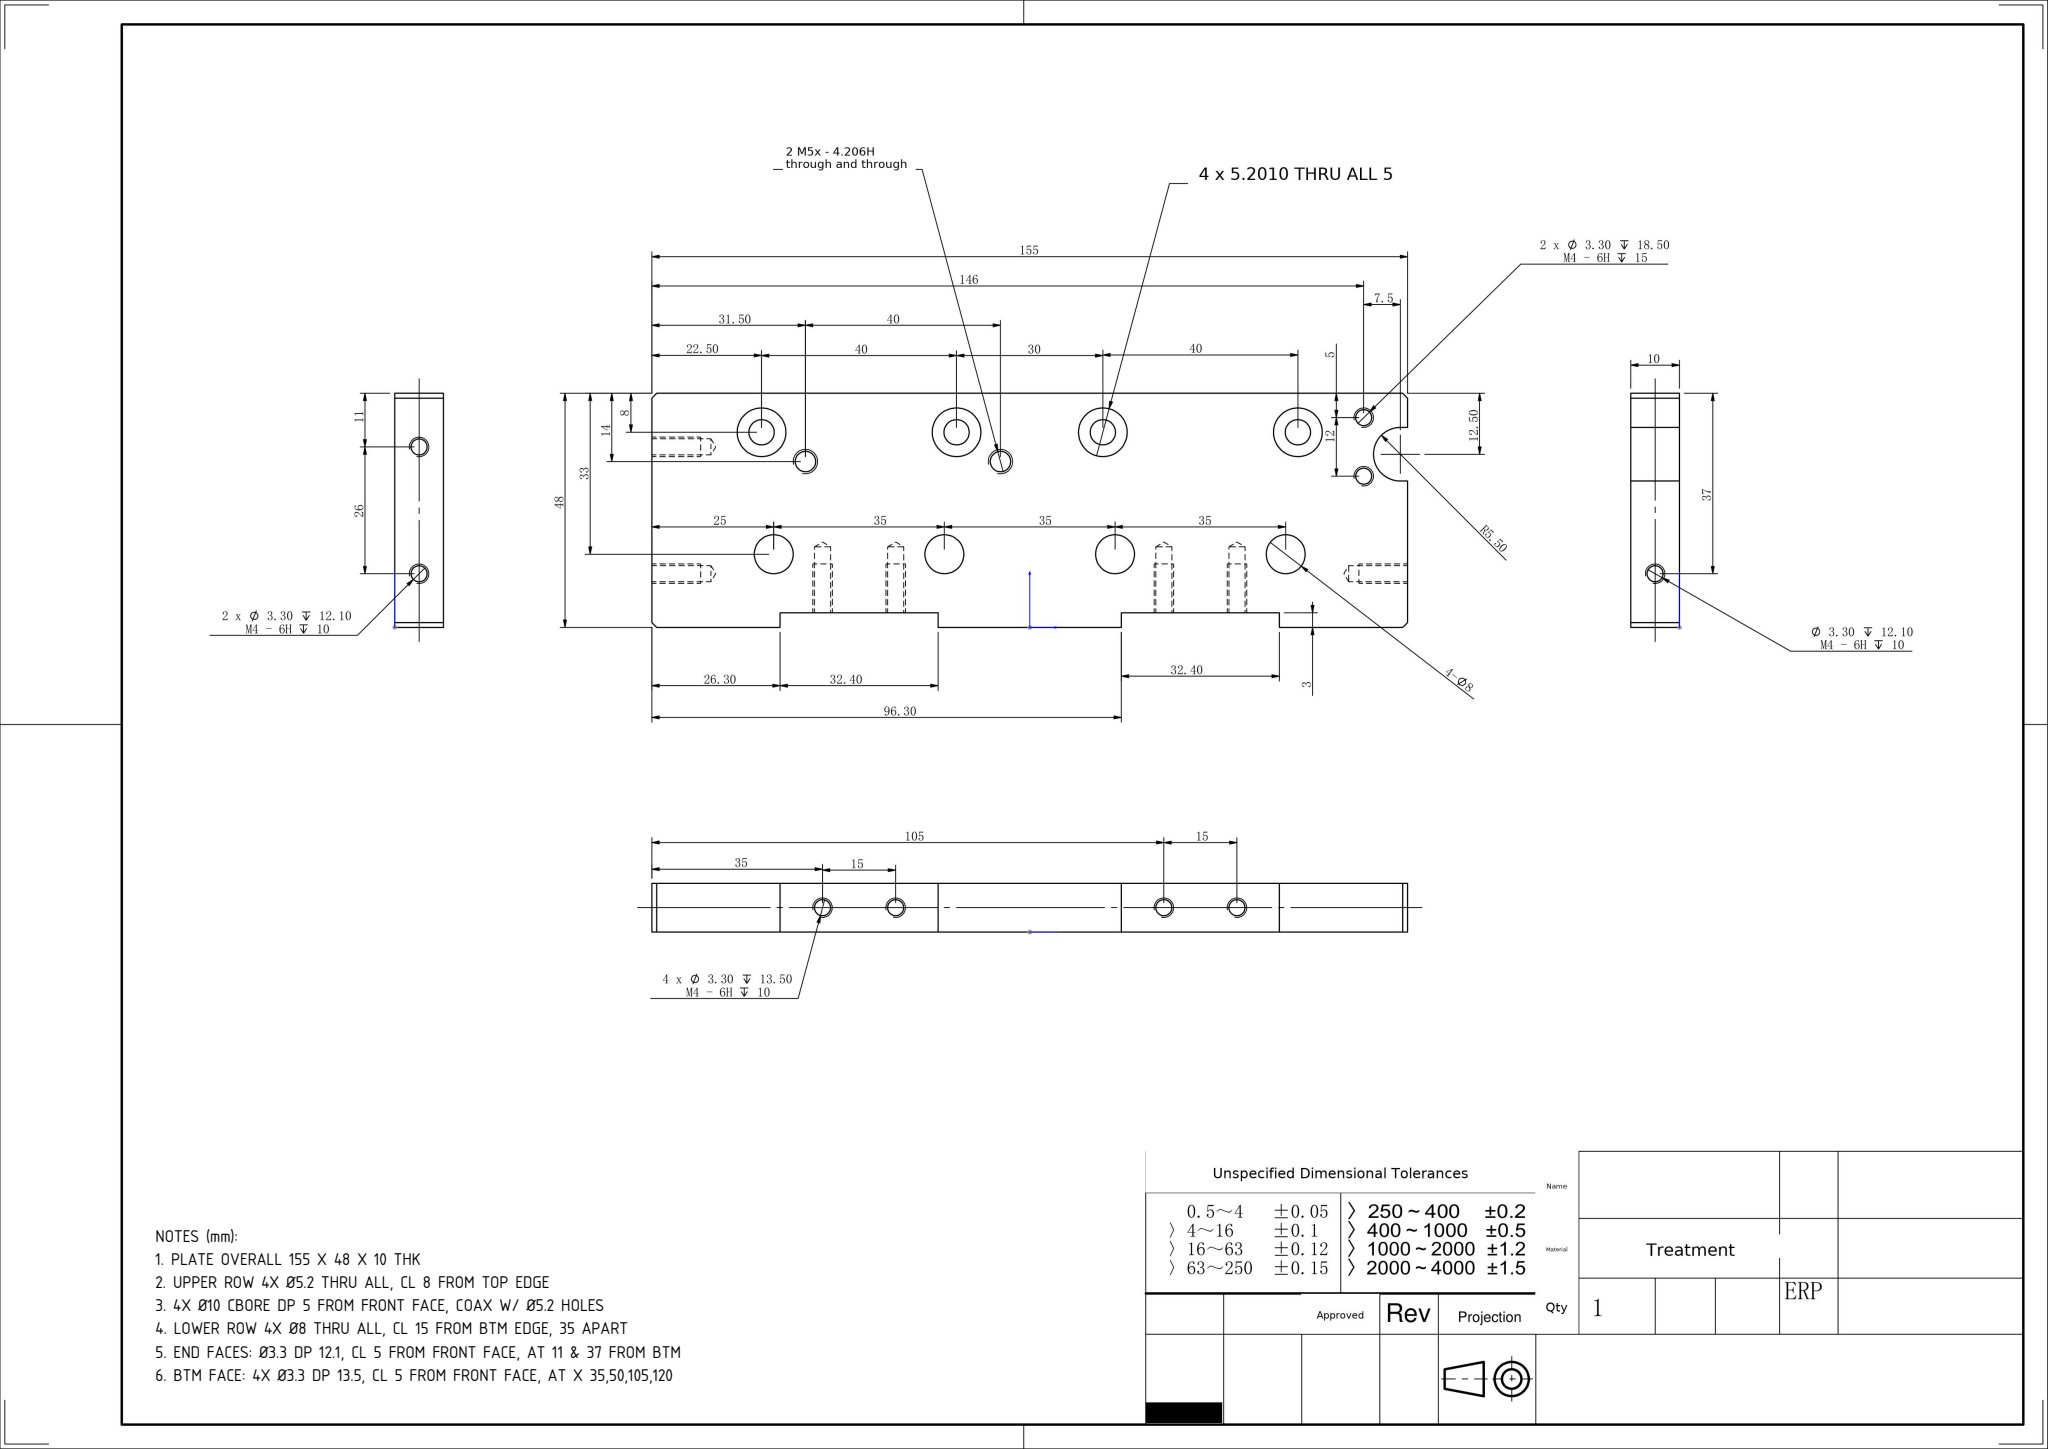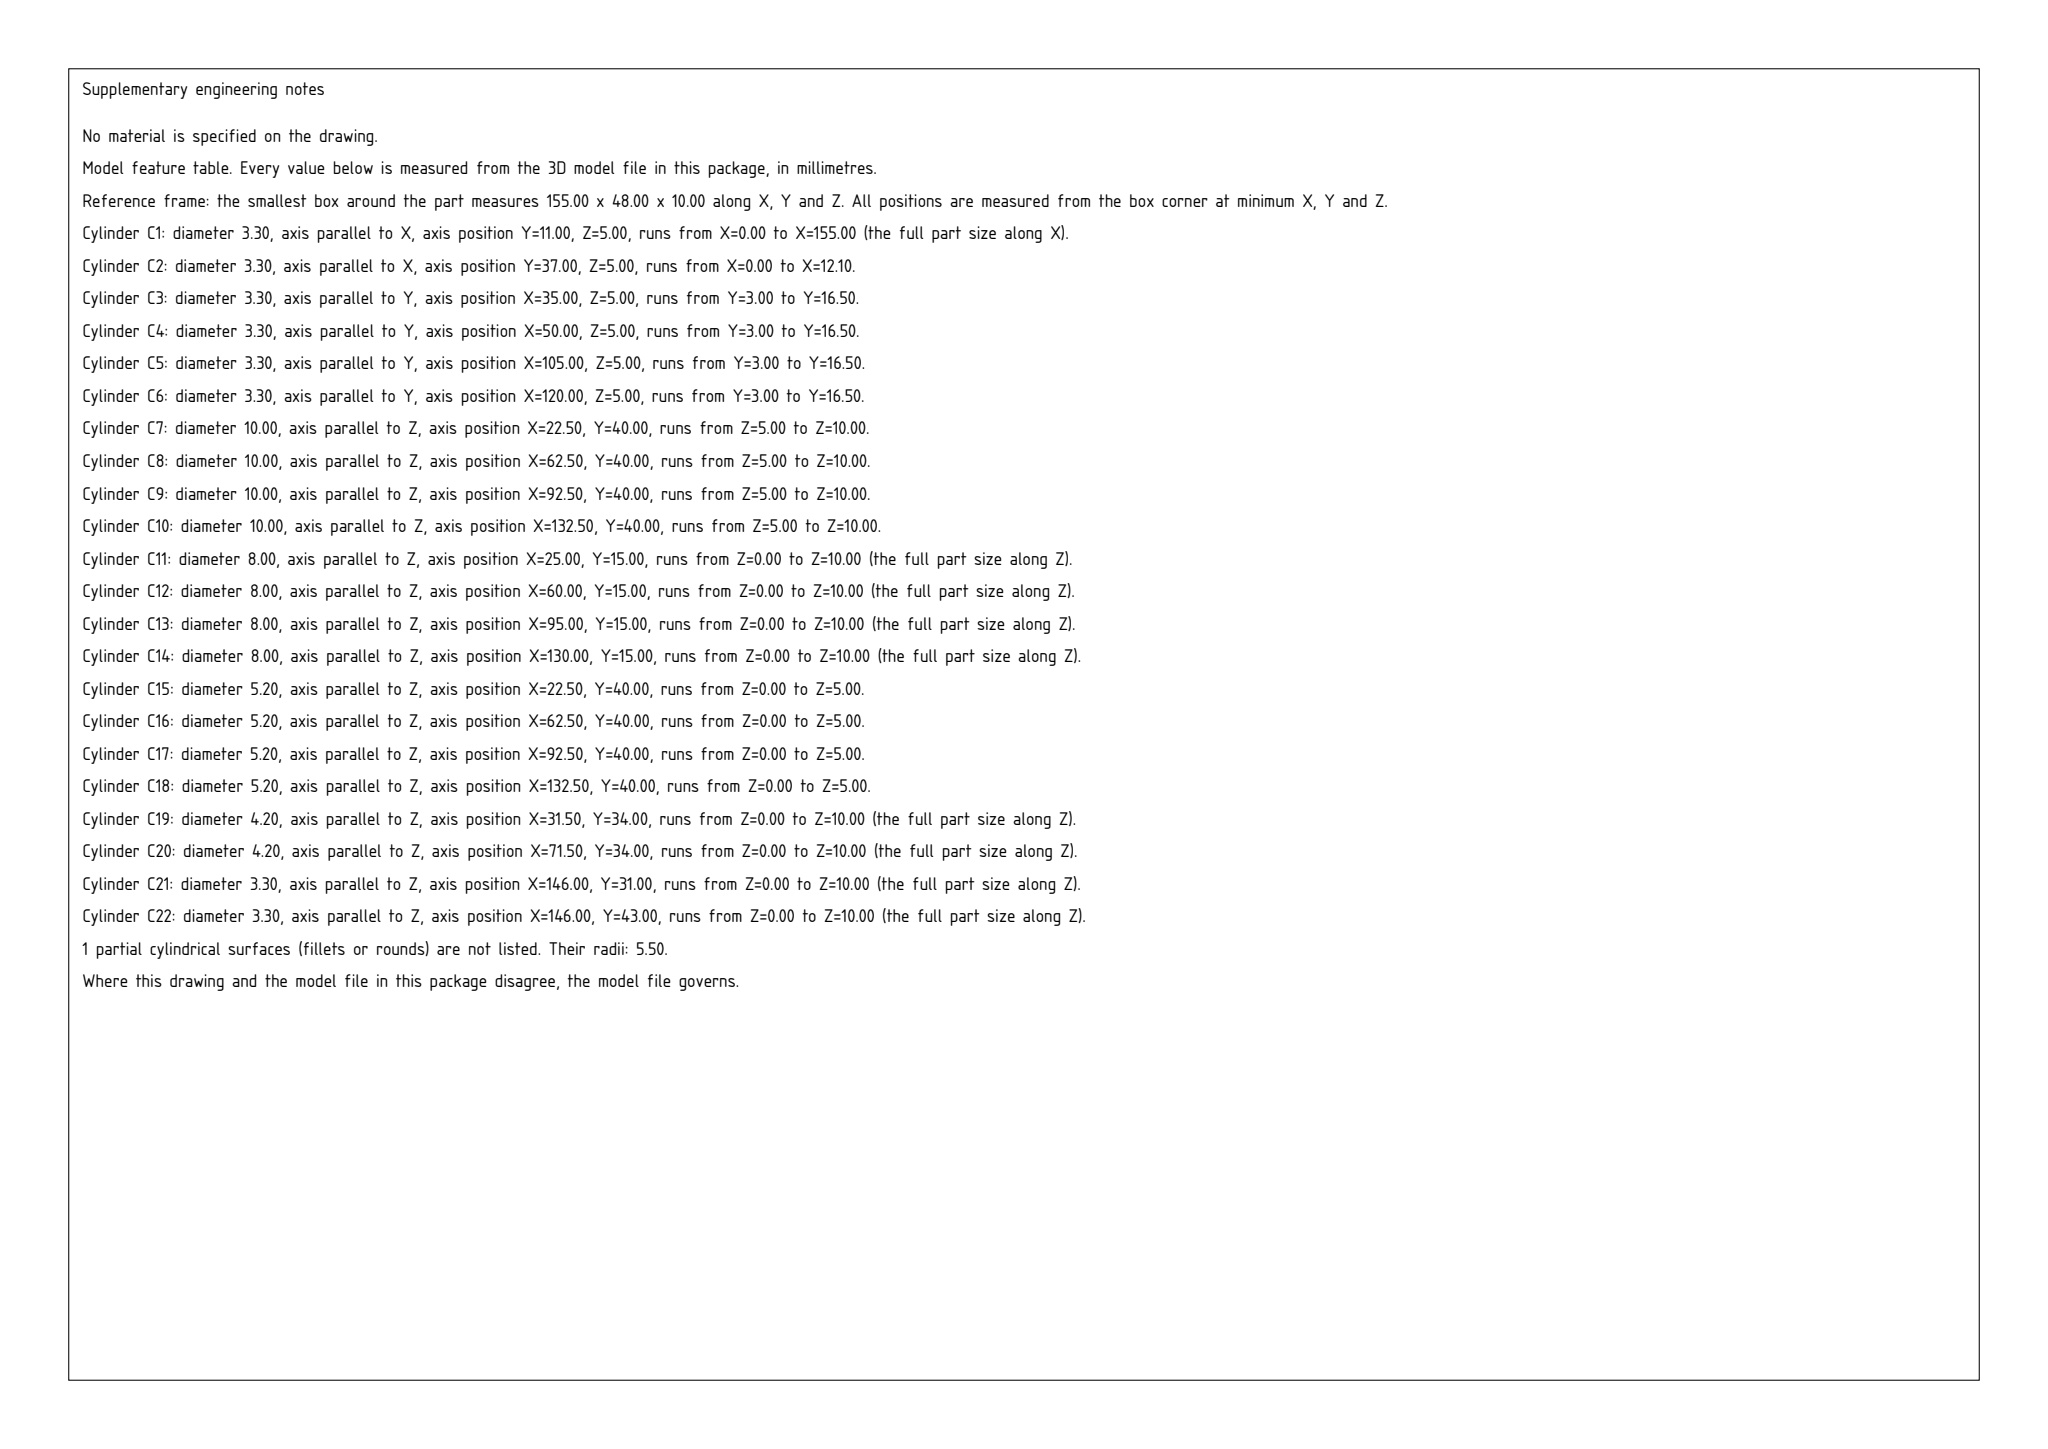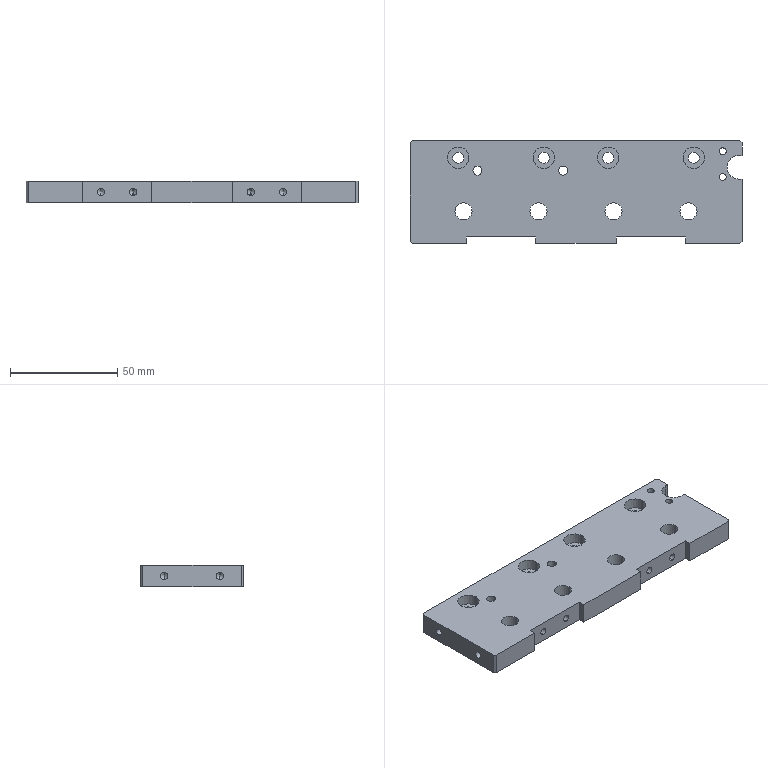Part | SolidWorks | mm | 1 solid | 86 faces | box 155 x 48 x 10 mm | volume 66549 mm3 | cylinder 47 | plane 25 | cone 14 | commonest cylinder face diameters 3.3 x18 8 x8 10 x8 5.2 x8 4.2 x4 11 x1
Drawing notes:
PLATE OVERALL 155 X 48 X 10 THK | from the solid: bbox_xyz 155,48,10
UPPER ROW 4X Ø5.2 THRU ALL, CL 8 FROM TOP EDGE | from the solid: cyl dia 5.2 axis z at (22.5,40),(62.5,40),(92.5,40),(132.5,40); bbox Y=48
4X Ø10 CBORE DP 5 FROM FRONT FACE, COAX W/ Ø5.2 HOLES | from the solid: cyl dia 10.0 axis z len 5 at same XY as Ø5.2 holes; plate thk 10
LOWER ROW 4X Ø8 THRU ALL, CL 15 FROM BTM EDGE, 35 APART | from the solid: cyl dia 8.0 axis z len 10 at (25,15),(60,15),(95,15),(130,15)
END FACES: Ø3.3 DP 12.1, CL 5 FROM FRONT FACE, AT 11 & 37 FROM BTM | from the solid: cyl 3.3 axis x at y=11 and y=37, z=5, L=12.1
BTM FACE: 4X Ø3.3 DP 13.5, CL 5 FROM FRONT FACE, AT X 35,50,105,120 | from the solid: cyl 3.3 axis y at x=35,50,105,120, z=5, L=13.5
build123d program:
from build123d import *

# Parameters (mm, degrees)
SKETCH1_W                                       = 155
SKETCH1_H                                       = 48
BOSS_EXTRUDE1_DEPTH                             = 10
M5_HEX_SOCKET_HEAD_CAP_SCREW_CBORE1_D           = 5.2
M5_HEX_SOCKET_HEAD_CAP_SCREW_CBORE1_CBORE_D     = 10
M5_HEX_SOCKET_HEAD_CAP_SCREW_CBORE1_CBORE_DEPTH = 5
SKETCH3_R                                       = 4
CUT_EXTRUDE1_DEPTH                              = 92.707
LPATTERN1_COUNT                                 = 4
LPATTERN1_PITCH                                 = 35
M4_TAPPED_HOLE2_D                               = 3.3
M4_TAPPED_HOLE2_DEPTH                           = 18.5
M4_TAPPED_HOLE2_TIP                             = 0.9914
SKETCH9_W                                       = 32.4
SKETCH9_H                                       = 44.674
CUT_EXTRUDE4_DEPTH                              = 3
M4_TAPPED_HOLE3_AT_2_COUNT                      = 2
M4_TAPPED_HOLE3_AT_2_PITCH                      = 15
LPATTERN2_COUNT                                 = 2
LPATTERN2_PITCH                                 = 70
CHAMFER1_SIZE                                   = 1
M5_TAPPED_HOLE2_D                               = 4.2
CUT_EXTRUDE5_DEPTH                              = 92.707
M4_TAPPED_HOLE4_D                               = 3.3
M4_TAPPED_HOLE4_DEPTH                           = 12.1
M4_TAPPED_HOLE4_TIP                             = 0.9914
M4_TAPPED_HOLE5_D                               = 3.3
M4_TAPPED_HOLE5_DEPTH                           = 12.1
M4_TAPPED_HOLE5_TIP                             = 0.9914


with BuildPart() as part:
    # Sketch1 → Boss-Extrude1 (new body)
    with BuildSketch(Plane.XY):
        with Locations((0, 24)):
            Rectangle(SKETCH1_W, SKETCH1_H)
    extrude(amount=BOSS_EXTRUDE1_DEPTH)

    # M5 Hex Socket Head Cap Screw CBORE1 (through all)
    with Locations(Plane(origin=(-55, 40, 10), x_dir=(1, 0, 0), z_dir=(0, 0, 1))):
        with Locations((0, 0), (40, 0), (70, 0), (110, 0)):
            CounterBoreHole(M5_HEX_SOCKET_HEAD_CAP_SCREW_CBORE1_D / 2, M5_HEX_SOCKET_HEAD_CAP_SCREW_CBORE1_CBORE_D / 2, M5_HEX_SOCKET_HEAD_CAP_SCREW_CBORE1_CBORE_DEPTH)

    # Sketch3 → Cut-Extrude1 (cut, through all)
    with BuildSketch(Plane.XY.offset(10)):
        with Locations((-52.5, 15)):
            Circle(SKETCH3_R)
    cut_extrude1 = extrude(amount=-CUT_EXTRUDE1_DEPTH, mode=Mode.SUBTRACT)

    # LPattern1: Cut-Extrude1 ×4
    with Locations(*[(i * LPATTERN1_PITCH, 0, 0) for i in range(1, LPATTERN1_COUNT)]):
        add(cut_extrude1, mode=Mode.SUBTRACT)

    # M4 Tapped Hole2
    with Locations(Plane(origin=(68.5, 31, 10), x_dir=(1, 0, 0), z_dir=(0, 0, 1))):
        with Locations((0, 0), (0, 12)):
            Hole(M4_TAPPED_HOLE2_D / 2, depth=M4_TAPPED_HOLE2_DEPTH)
            with Locations((0, 0, -(M4_TAPPED_HOLE2_DEPTH + M4_TAPPED_HOLE2_TIP / 2))):  # 118° drill point
                Cone(0, M4_TAPPED_HOLE2_D / 2, M4_TAPPED_HOLE2_TIP, mode=Mode.SUBTRACT)

    # Sketch9 → Cut-Extrude4 (cut)
    with BuildSketch(Plane.XZ):
        with Locations((-35, 3.88)):
            Rectangle(SKETCH9_W, SKETCH9_H)
    cut_extrude4 = extrude(amount=-CUT_EXTRUDE4_DEPTH, mode=Mode.SUBTRACT)

    # Sketch10 → M4 Tapped Hole3 (revolve, cut)
    with BuildSketch(Plane(origin=(-42.5, 3, 5), x_dir=(0, 0, -1), z_dir=(1, 0, 0))):
        Polygon((0, 0), (0, 14.491), (1.65, 13.5), (1.65, 0), align=None)
    m4_tapped_hole3 = revolve(axis=Axis((-42.5, -3.35, 5), (0, 1, 0)), mode=Mode.SUBTRACT)

    # M4 Tapped Hole3 at 2: M4 Tapped Hole3 ×2
    with Locations(*[(i * M4_TAPPED_HOLE3_AT_2_PITCH, 0, 0) for i in range(1, M4_TAPPED_HOLE3_AT_2_COUNT)]):
        add(m4_tapped_hole3, mode=Mode.SUBTRACT)

    # LPattern2: Cut-Extrude4, M4 Tapped Hole3 ×2
    with Locations(*[(i * LPATTERN2_PITCH, 0, 0) for i in range(1, LPATTERN2_COUNT)]):
        add(cut_extrude4, mode=Mode.SUBTRACT)
        add(m4_tapped_hole3, mode=Mode.SUBTRACT)

    # LPattern2 copy 1 sketch → LPattern2 copy 1 (revolve, cut)
    with BuildSketch(Plane(origin=(42.5, 3, 5), x_dir=(0, 0, -1), z_dir=(1, 0, 0))):
        Polygon((0, 0), (0, 14.491), (1.65, 13.5), (1.65, 0), align=None)
    revolve(axis=Axis((42.5, -3.35, 5), (0, 1, 0)), mode=Mode.SUBTRACT)

    # Chamfer1
    chamfer1_edges = [part.edges().sort_by_distance(p)[0] for p in [
        (-77.5, 48, 5),
        (77.5, 48, 5),
        (77.5, 0, 5),
        (-77.5, 0, 5),
    ]]
    chamfer(chamfer1_edges, length=CHAMFER1_SIZE)

    # M5 Tapped Hole2 (through all)
    with Locations(Plane(origin=(-46, 34, 10), x_dir=(1, 0, 0), z_dir=(0, 0, 1))):
        with Locations((0, 0), (40, 0)):
            Hole(M5_TAPPED_HOLE2_D / 2)

    # Sketch12 → Cut-Extrude5 (cut, through all)
    with BuildSketch(Plane.XY.offset(10)):
        with BuildLine():
            Line((76, 41), (86.024, 41))
            Line((86.024, 41), (86.024, 30))
            Line((86.024, 30), (76, 30))
            ThreePointArc((76, 30), (70.5, 35.5), (76, 41))
        make_face()
    extrude(amount=-CUT_EXTRUDE5_DEPTH, mode=Mode.SUBTRACT)

    # M4 Tapped Hole4
    with Locations(Plane(origin=(-77.5, 11, 5), x_dir=(0, 0, -1), z_dir=(-1, 0, 0))):
        with Locations((0, 0), (0, -26)):
            Hole(M4_TAPPED_HOLE4_D / 2, depth=M4_TAPPED_HOLE4_DEPTH)
            with Locations((0, 0, -(M4_TAPPED_HOLE4_DEPTH + M4_TAPPED_HOLE4_TIP / 2))):  # 118° drill point
                Cone(0, M4_TAPPED_HOLE4_D / 2, M4_TAPPED_HOLE4_TIP, mode=Mode.SUBTRACT)

    # M4 Tapped Hole5
    with Locations(Plane(origin=(77.5, 11, 5), x_dir=(0, 0, 1), z_dir=(1, 0, 0))):
        with Locations((0, 0)):
            Hole(M4_TAPPED_HOLE5_D / 2, depth=M4_TAPPED_HOLE5_DEPTH)
            with Locations((0, 0, -(M4_TAPPED_HOLE5_DEPTH + M4_TAPPED_HOLE5_TIP / 2))):  # 118° drill point
                Cone(0, M4_TAPPED_HOLE5_D / 2, M4_TAPPED_HOLE5_TIP, mode=Mode.SUBTRACT)


solid = part.part